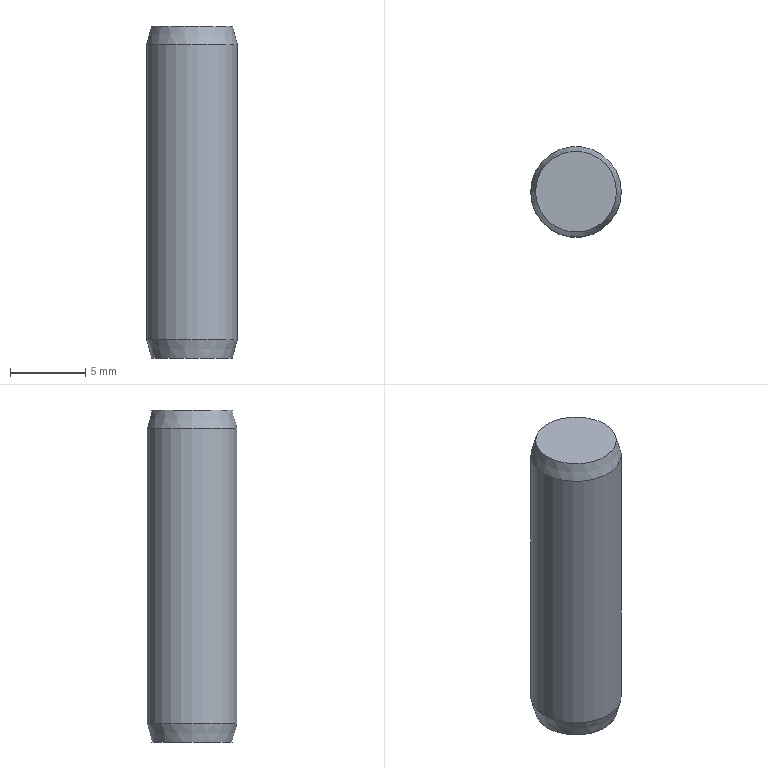Component | NX | GB-T119_1-2000_6X22 | 1 solid | 5 faces | box 6 x 6 x 22 mm | volume 615 mm3 | plane 2 | cone 2 | cylinder 1 | commonest cylinder face diameters 6 x1
STEP:
#1=CARTESIAN_POINT('',(0.,0.,0.));
#2=DIRECTION('',(0.,0.,1.));
#3=DIRECTION('',(1.,0.,0.));
#4=AXIS2_PLACEMENT_3D('',#1,#2,#3);
#5=CARTESIAN_POINT('',(9.322,81.,-110.));
#6=VERTEX_POINT('',#5);
#7=CARTESIAN_POINT('',(12.,81.,-110.));
#8=DIRECTION('',(0.,0.,-1.));
#9=DIRECTION('',(-1.,0.,0.));
#10=AXIS2_PLACEMENT_3D('',#7,#8,#9);
#11=CIRCLE('',#10,2.678);
#12=CARTESIAN_POINT('',(12.,81.,-110.));
#13=DIRECTION('',(0.,0.,-1.));
#14=DIRECTION('',(-1.,0.,0.));
#15=AXIS2_PLACEMENT_3D('',#12,#13,#14);
#16=PLANE('',#15);
#17=CARTESIAN_POINT('',(0.,0.));
#18=DIRECTION('',(1.,0.));
#19=AXIS2_PLACEMENT_2D('',#17,#18);
#20=CIRCLE('',#19,2.678);
#21=(GEOMETRIC_REPRESENTATION_CONTEXT(2)PARAMETRIC_REPRESENTATION_CONTEXT()REPRESENTATION_CONTEXT('',''));
#22=DEFINITIONAL_REPRESENTATION('',(#20),#21);
#23=PCURVE('',#16,#22);
#24=CARTESIAN_POINT('',(12.,81.,-110.));
#25=DIRECTION('',(0.,0.,1.));
#26=DIRECTION('',(1.,0.,0.));
#27=AXIS2_PLACEMENT_3D('',#24,#25,#26);
#28=CONICAL_SURFACE('',#27,2.678,0.2618);
#29=CARTESIAN_POINT('',(9.425,0.));
#30=DIRECTION('',(-1.,0.));
#31=VECTOR('',#30,1.);
#32=LINE('',#29,#31);
#33=(GEOMETRIC_REPRESENTATION_CONTEXT(2)PARAMETRIC_REPRESENTATION_CONTEXT()REPRESENTATION_CONTEXT('',''));
#34=DEFINITIONAL_REPRESENTATION('',(#32),#33);
#35=PCURVE('',#28,#34);
#36=SURFACE_CURVE('',#11,(#23,#35),.PCURVE_S1.);
#37=EDGE_CURVE('',#6,#6,#36,.T.);
#38=ORIENTED_EDGE('',*,*,#37,.T.);
#39=EDGE_LOOP('',(#38));
#40=FACE_BOUND('',#39,.T.);
#41=ADVANCED_FACE('',(#40),#16,.T.);
#42=CARTESIAN_POINT('',(9.,81.,-108.8));
#43=VERTEX_POINT('',#42);
#44=CARTESIAN_POINT('',(12.,81.,-108.8));
#45=DIRECTION('',(0.,0.,-1.));
#46=DIRECTION('',(-1.,0.,0.));
#47=AXIS2_PLACEMENT_3D('',#44,#45,#46);
#48=CIRCLE('',#47,3.);
#49=CARTESIAN_POINT('',(9.425,1.2));
#50=DIRECTION('',(-1.,0.));
#51=VECTOR('',#50,1.);
#52=LINE('',#49,#51);
#53=(GEOMETRIC_REPRESENTATION_CONTEXT(2)PARAMETRIC_REPRESENTATION_CONTEXT()REPRESENTATION_CONTEXT('',''));
#54=DEFINITIONAL_REPRESENTATION('',(#52),#53);
#55=PCURVE('',#28,#54);
#56=CARTESIAN_POINT('',(12.,81.,-88.));
#57=DIRECTION('',(0.,0.,-1.));
#58=DIRECTION('',(-1.,0.,0.));
#59=AXIS2_PLACEMENT_3D('',#56,#57,#58);
#60=CYLINDRICAL_SURFACE('',#59,3.);
#61=CARTESIAN_POINT('',(0.,20.8));
#62=DIRECTION('',(1.,0.));
#63=VECTOR('',#62,1.);
#64=LINE('',#61,#63);
#65=(GEOMETRIC_REPRESENTATION_CONTEXT(2)PARAMETRIC_REPRESENTATION_CONTEXT()REPRESENTATION_CONTEXT('',''));
#66=DEFINITIONAL_REPRESENTATION('',(#64),#65);
#67=PCURVE('',#60,#66);
#68=SURFACE_CURVE('',#48,(#55,#67),.PCURVE_S1.);
#69=EDGE_CURVE('',#43,#43,#68,.T.);
#70=ORIENTED_EDGE('',*,*,#69,.T.);
#71=CARTESIAN_POINT('',(9.322,81.,-110.));
#72=CARTESIAN_POINT('',(9.,81.,-108.8));
#73=B_SPLINE_CURVE_WITH_KNOTS('',1,(#71,#72),.UNSPECIFIED.,.F.,.F.,(2,2),(0.,1.242),.PIECEWISE_BEZIER_KNOTS.);
#74=CARTESIAN_POINT('',(3.142,0.));
#75=DIRECTION('',(0.,1.));
#76=VECTOR('',#75,1.);
#77=LINE('',#74,#76);
#78=(GEOMETRIC_REPRESENTATION_CONTEXT(2)PARAMETRIC_REPRESENTATION_CONTEXT()REPRESENTATION_CONTEXT('',''));
#79=DEFINITIONAL_REPRESENTATION('',(#77),#78);
#80=PCURVE('',#28,#79);
#81=CARTESIAN_POINT('',(9.425,0.));
#82=DIRECTION('',(0.,1.));
#83=VECTOR('',#82,1.);
#84=LINE('',#81,#83);
#85=(GEOMETRIC_REPRESENTATION_CONTEXT(2)PARAMETRIC_REPRESENTATION_CONTEXT()REPRESENTATION_CONTEXT('',''));
#86=DEFINITIONAL_REPRESENTATION('',(#84),#85);
#87=PCURVE('',#28,#86);
#88=SEAM_CURVE('',#73,(#80,#87),.PCURVE_S1.);
#89=EDGE_CURVE('',#6,#43,#88,.T.);
#90=ORIENTED_EDGE('',*,*,#89,.F.);
#91=ORIENTED_EDGE('',*,*,#37,.F.);
#92=ORIENTED_EDGE('',*,*,#89,.T.);
#93=EDGE_LOOP('',(#70,#90,#91,#92));
#94=FACE_BOUND('',#93,.T.);
#95=ADVANCED_FACE('',(#94),#28,.T.);
#96=CARTESIAN_POINT('',(9.,81.,-89.2));
#97=VERTEX_POINT('',#96);
#98=CARTESIAN_POINT('',(12.,81.,-89.2));
#99=DIRECTION('',(0.,0.,-1.));
#100=DIRECTION('',(-1.,0.,0.));
#101=AXIS2_PLACEMENT_3D('',#98,#99,#100);
#102=CIRCLE('',#101,3.);
#103=CARTESIAN_POINT('',(0.,1.2));
#104=DIRECTION('',(1.,0.));
#105=VECTOR('',#104,1.);
#106=LINE('',#103,#105);
#107=(GEOMETRIC_REPRESENTATION_CONTEXT(2)PARAMETRIC_REPRESENTATION_CONTEXT()REPRESENTATION_CONTEXT('',''));
#108=DEFINITIONAL_REPRESENTATION('',(#106),#107);
#109=PCURVE('',#60,#108);
#110=CARTESIAN_POINT('',(12.,81.,-89.2));
#111=DIRECTION('',(0.,0.,-1.));
#112=DIRECTION('',(-1.,0.,0.));
#113=AXIS2_PLACEMENT_3D('',#110,#111,#112);
#114=CONICAL_SURFACE('',#113,3.,0.2618);
#115=CARTESIAN_POINT('',(0.,0.));
#116=DIRECTION('',(1.,0.));
#117=VECTOR('',#116,1.);
#118=LINE('',#115,#117);
#119=(GEOMETRIC_REPRESENTATION_CONTEXT(2)PARAMETRIC_REPRESENTATION_CONTEXT()REPRESENTATION_CONTEXT('',''));
#120=DEFINITIONAL_REPRESENTATION('',(#118),#119);
#121=PCURVE('',#114,#120);
#122=SURFACE_CURVE('',#102,(#109,#121),.PCURVE_S1.);
#123=EDGE_CURVE('',#97,#97,#122,.T.);
#124=ORIENTED_EDGE('',*,*,#123,.T.);
#125=CARTESIAN_POINT('',(9.,81.,-89.2));
#126=CARTESIAN_POINT('',(9.,81.,-108.8));
#127=B_SPLINE_CURVE_WITH_KNOTS('',1,(#125,#126),.UNSPECIFIED.,.F.,.F.,(2,2),(1.2,20.8),.PIECEWISE_BEZIER_KNOTS.);
#128=CARTESIAN_POINT('',(6.283,0.));
#129=DIRECTION('',(0.,1.));
#130=VECTOR('',#129,1.);
#131=LINE('',#128,#130);
#132=(GEOMETRIC_REPRESENTATION_CONTEXT(2)PARAMETRIC_REPRESENTATION_CONTEXT()REPRESENTATION_CONTEXT('',''));
#133=DEFINITIONAL_REPRESENTATION('',(#131),#132);
#134=PCURVE('',#60,#133);
#135=CARTESIAN_POINT('',(0.,0.));
#136=DIRECTION('',(0.,1.));
#137=VECTOR('',#136,1.);
#138=LINE('',#135,#137);
#139=(GEOMETRIC_REPRESENTATION_CONTEXT(2)PARAMETRIC_REPRESENTATION_CONTEXT()REPRESENTATION_CONTEXT('',''));
#140=DEFINITIONAL_REPRESENTATION('',(#138),#139);
#141=PCURVE('',#60,#140);
#142=SEAM_CURVE('',#127,(#134,#141),.PCURVE_S1.);
#143=EDGE_CURVE('',#97,#43,#142,.T.);
#144=ORIENTED_EDGE('',*,*,#143,.T.);
#145=ORIENTED_EDGE('',*,*,#69,.F.);
#146=ORIENTED_EDGE('',*,*,#143,.F.);
#147=EDGE_LOOP('',(#124,#144,#145,#146));
#148=FACE_BOUND('',#147,.T.);
#149=ADVANCED_FACE('',(#148),#60,.T.);
#150=CARTESIAN_POINT('',(9.322,81.,-88.));
#151=VERTEX_POINT('',#150);
#152=CARTESIAN_POINT('',(12.,81.,-88.));
#153=DIRECTION('',(0.,0.,-1.));
#154=DIRECTION('',(-1.,0.,0.));
#155=AXIS2_PLACEMENT_3D('',#152,#153,#154);
#156=CIRCLE('',#155,2.678);
#157=CARTESIAN_POINT('',(0.,-1.2));
#158=DIRECTION('',(1.,0.));
#159=VECTOR('',#158,1.);
#160=LINE('',#157,#159);
#161=(GEOMETRIC_REPRESENTATION_CONTEXT(2)PARAMETRIC_REPRESENTATION_CONTEXT()REPRESENTATION_CONTEXT('',''));
#162=DEFINITIONAL_REPRESENTATION('',(#160),#161);
#163=PCURVE('',#114,#162);
#164=CARTESIAN_POINT('',(14.678,81.,-88.));
#165=DIRECTION('',(0.,0.,1.));
#166=DIRECTION('',(1.,0.,0.));
#167=AXIS2_PLACEMENT_3D('',#164,#165,#166);
#168=PLANE('',#167);
#169=CARTESIAN_POINT('',(-5.357,0.));
#170=CARTESIAN_POINT('',(-5.357,4.639));
#171=CARTESIAN_POINT('',(-1.339,2.32));
#172=CARTESIAN_POINT('',(2.678,0.));
#173=CARTESIAN_POINT('',(-1.339,-2.32));
#174=CARTESIAN_POINT('',(-5.357,-4.639));
#175=CARTESIAN_POINT('',(-5.357,0.));
#176=(BOUNDED_CURVE()B_SPLINE_CURVE(2,(#169,#170,#171,#172,#173,#174,#175),.UNSPECIFIED.,.T.,.F.)B_SPLINE_CURVE_WITH_KNOTS((1,2,2,2,2,1),(-2.094,0.,2.094,4.189,6.283,8.378),.UNSPECIFIED.)CURVE()GEOMETRIC_REPRESENTATION_ITEM()RATIONAL_B_SPLINE_CURVE((1.,0.5,1.,0.5,1.,0.5,1.))REPRESENTATION_ITEM(''));
#177=(GEOMETRIC_REPRESENTATION_CONTEXT(2)PARAMETRIC_REPRESENTATION_CONTEXT()REPRESENTATION_CONTEXT('',''));
#178=DEFINITIONAL_REPRESENTATION('',(#176),#177);
#179=PCURVE('',#168,#178);
#180=SURFACE_CURVE('',#156,(#163,#179),.PCURVE_S1.);
#181=EDGE_CURVE('',#151,#151,#180,.T.);
#182=ORIENTED_EDGE('',*,*,#181,.T.);
#183=CARTESIAN_POINT('',(9.322,81.,-88.));
#184=CARTESIAN_POINT('',(9.,81.,-89.2));
#185=B_SPLINE_CURVE_WITH_KNOTS('',1,(#183,#184),.UNSPECIFIED.,.F.,.F.,(2,2),(-1.242,0.),.PIECEWISE_BEZIER_KNOTS.);
#186=CARTESIAN_POINT('',(6.283,0.));
#187=DIRECTION('',(0.,1.));
#188=VECTOR('',#187,1.);
#189=LINE('',#186,#188);
#190=(GEOMETRIC_REPRESENTATION_CONTEXT(2)PARAMETRIC_REPRESENTATION_CONTEXT()REPRESENTATION_CONTEXT('',''));
#191=DEFINITIONAL_REPRESENTATION('',(#189),#190);
#192=PCURVE('',#114,#191);
#193=CARTESIAN_POINT('',(0.,0.));
#194=DIRECTION('',(0.,1.));
#195=VECTOR('',#194,1.);
#196=LINE('',#193,#195);
#197=(GEOMETRIC_REPRESENTATION_CONTEXT(2)PARAMETRIC_REPRESENTATION_CONTEXT()REPRESENTATION_CONTEXT('',''));
#198=DEFINITIONAL_REPRESENTATION('',(#196),#197);
#199=PCURVE('',#114,#198);
#200=SEAM_CURVE('',#185,(#192,#199),.PCURVE_S1.);
#201=EDGE_CURVE('',#151,#97,#200,.T.);
#202=ORIENTED_EDGE('',*,*,#201,.T.);
#203=ORIENTED_EDGE('',*,*,#123,.F.);
#204=ORIENTED_EDGE('',*,*,#201,.F.);
#205=EDGE_LOOP('',(#182,#202,#203,#204));
#206=FACE_BOUND('',#205,.T.);
#207=ADVANCED_FACE('',(#206),#114,.T.);
#208=ORIENTED_EDGE('',*,*,#181,.F.);
#209=EDGE_LOOP('',(#208));
#210=FACE_BOUND('',#209,.T.);
#211=ADVANCED_FACE('',(#210),#168,.T.);
#212=CLOSED_SHELL('',(#41,#95,#149,#207,#211));
#213=MANIFOLD_SOLID_BREP('',#212);
#214=(LENGTH_UNIT()NAMED_UNIT(*)SI_UNIT(.MILLI.,.METRE.));
#215=UNCERTAINTY_MEASURE_WITH_UNIT(LENGTH_MEASURE(0.00001),#214,'','');
#216=(NAMED_UNIT(*)PLANE_ANGLE_UNIT()SI_UNIT($,.RADIAN.));
#217=(NAMED_UNIT(*)SI_UNIT($,.STERADIAN.)SOLID_ANGLE_UNIT());
#218=(GEOMETRIC_REPRESENTATION_CONTEXT(3)GLOBAL_UNCERTAINTY_ASSIGNED_CONTEXT((#215))GLOBAL_UNIT_ASSIGNED_CONTEXT((#214,#216,#217))REPRESENTATION_CONTEXT('',''));
#219=ADVANCED_BREP_SHAPE_REPRESENTATION('',(#4,#213),#218);